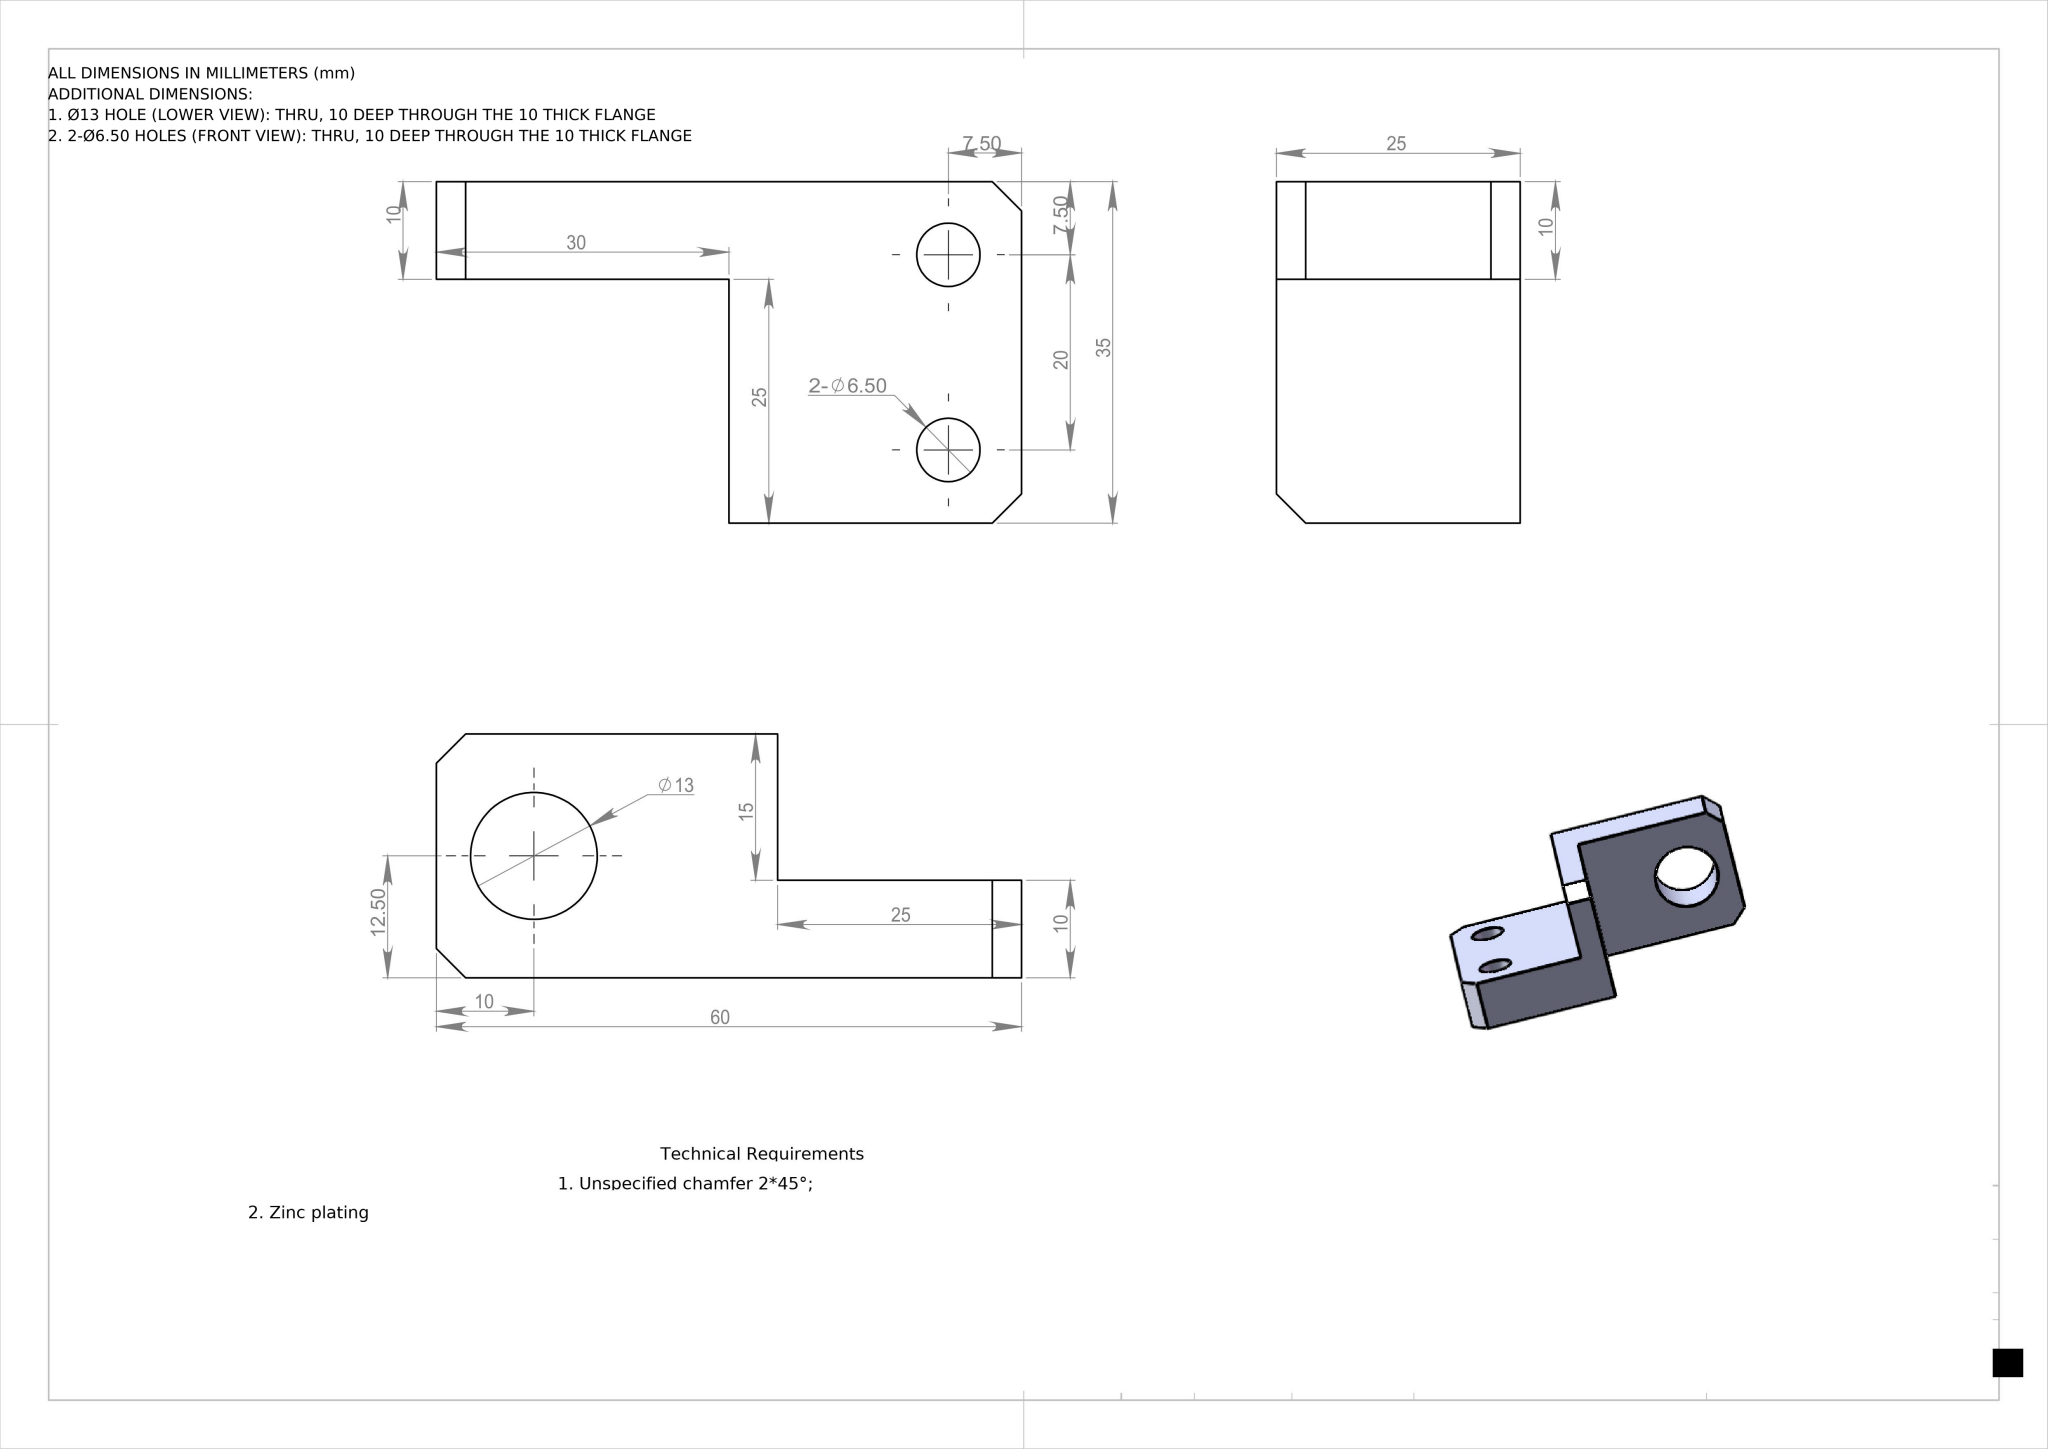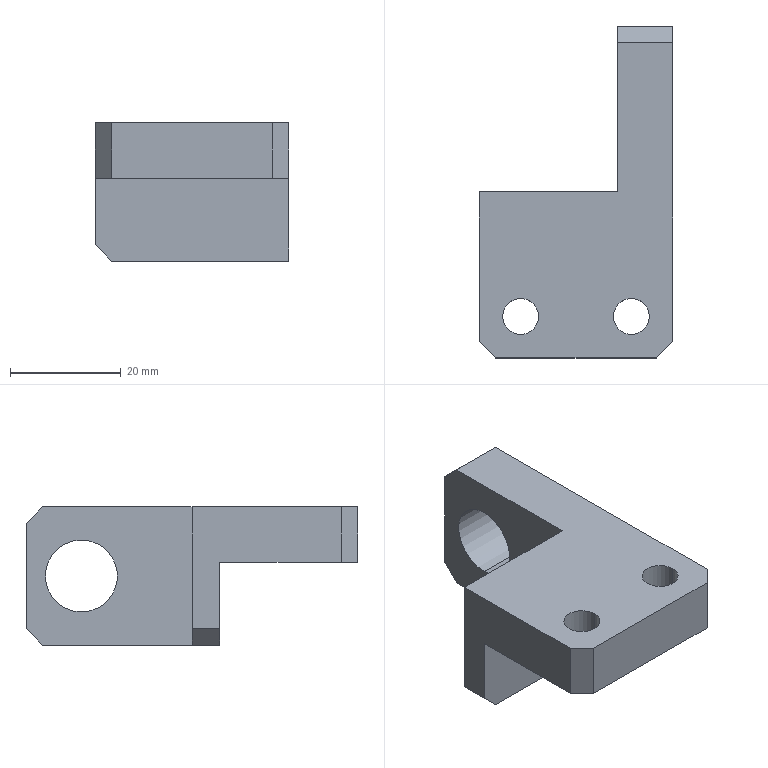Part | NX | mm | 1 solid | 21 faces | box 35 x 60 x 25 mm | volume 18432 mm3 | plane 15 | cylinder 6 | commonest cylinder face diameters 6.5 x4 13 x2
STEP:
#1=COLOUR_RGB('',0.7961,0.8235,0.9373);
#2=FILL_AREA_STYLE_COLOUR('',#1);
#3=FILL_AREA_STYLE('',(#2));
#4=SURFACE_STYLE_FILL_AREA(#3);
#5=SURFACE_SIDE_STYLE('',(#4));
#6=SURFACE_STYLE_USAGE(.BOTH.,#5);
#7=PRESENTATION_STYLE_ASSIGNMENT((#6));
#8=CARTESIAN_POINT('',(-13.25,-22.5,15.));
#9=VERTEX_POINT('',#8);
#10=CARTESIAN_POINT('',(-6.75,-22.5,15.));
#11=VERTEX_POINT('',#10);
#12=CARTESIAN_POINT('',(-10.,-22.5,15.));
#13=DIRECTION('',(0.,0.,1.));
#14=DIRECTION('',(1.,0.,0.));
#15=AXIS2_PLACEMENT_3D('',#12,#13,#14);
#16=CIRCLE('',#15,3.25);
#17=EDGE_CURVE('',#9,#11,#16,.T.);
#18=ORIENTED_EDGE('',*,*,#17,.F.);
#19=CARTESIAN_POINT('',(-13.25,-22.5,25.));
#20=VERTEX_POINT('',#19);
#21=CARTESIAN_POINT('',(-13.25,-22.5,0.));
#22=DIRECTION('',(0.,0.,1.));
#23=VECTOR('',#22,1000.);
#24=LINE('',#21,#23);
#25=EDGE_CURVE('',#9,#20,#24,.T.);
#26=ORIENTED_EDGE('',*,*,#25,.T.);
#27=CARTESIAN_POINT('',(-6.75,-22.5,25.));
#28=VERTEX_POINT('',#27);
#29=CARTESIAN_POINT('',(-10.,-22.5,25.));
#30=DIRECTION('',(0.,0.,1.));
#31=DIRECTION('',(1.,0.,0.));
#32=AXIS2_PLACEMENT_3D('',#29,#30,#31);
#33=CIRCLE('',#32,3.25);
#34=EDGE_CURVE('',#20,#28,#33,.T.);
#35=ORIENTED_EDGE('',*,*,#34,.T.);
#36=CARTESIAN_POINT('',(-6.75,-22.5,0.));
#37=DIRECTION('',(0.,0.,1.));
#38=VECTOR('',#37,1000.);
#39=LINE('',#36,#38);
#40=EDGE_CURVE('',#11,#28,#39,.T.);
#41=ORIENTED_EDGE('',*,*,#40,.F.);
#42=EDGE_LOOP('',(#18,#26,#35,#41));
#43=FACE_OUTER_BOUND('',#42,.T.);
#44=CARTESIAN_POINT('',(-10.,-22.5,0.));
#45=DIRECTION('',(0.,0.,1.));
#46=DIRECTION('',(1.,0.,0.));
#47=AXIS2_PLACEMENT_3D('',#44,#45,#46);
#48=CYLINDRICAL_SURFACE('',#47,3.25);
#49=ADVANCED_FACE('',(#43),#48,.F.);
#50=CARTESIAN_POINT('',(6.75,-22.5,15.));
#51=VERTEX_POINT('',#50);
#52=CARTESIAN_POINT('',(13.25,-22.5,15.));
#53=VERTEX_POINT('',#52);
#54=CARTESIAN_POINT('',(10.,-22.5,15.));
#55=DIRECTION('',(0.,0.,1.));
#56=DIRECTION('',(1.,0.,0.));
#57=AXIS2_PLACEMENT_3D('',#54,#55,#56);
#58=CIRCLE('',#57,3.25);
#59=EDGE_CURVE('',#51,#53,#58,.T.);
#60=ORIENTED_EDGE('',*,*,#59,.F.);
#61=CARTESIAN_POINT('',(6.75,-22.5,25.));
#62=VERTEX_POINT('',#61);
#63=CARTESIAN_POINT('',(6.75,-22.5,0.));
#64=DIRECTION('',(0.,0.,1.));
#65=VECTOR('',#64,1000.);
#66=LINE('',#63,#65);
#67=EDGE_CURVE('',#51,#62,#66,.T.);
#68=ORIENTED_EDGE('',*,*,#67,.T.);
#69=CARTESIAN_POINT('',(13.25,-22.5,25.));
#70=VERTEX_POINT('',#69);
#71=CARTESIAN_POINT('',(10.,-22.5,25.));
#72=DIRECTION('',(0.,0.,1.));
#73=DIRECTION('',(1.,0.,0.));
#74=AXIS2_PLACEMENT_3D('',#71,#72,#73);
#75=CIRCLE('',#74,3.25);
#76=EDGE_CURVE('',#62,#70,#75,.T.);
#77=ORIENTED_EDGE('',*,*,#76,.T.);
#78=CARTESIAN_POINT('',(13.25,-22.5,0.));
#79=DIRECTION('',(0.,0.,1.));
#80=VECTOR('',#79,1000.);
#81=LINE('',#78,#80);
#82=EDGE_CURVE('',#53,#70,#81,.T.);
#83=ORIENTED_EDGE('',*,*,#82,.F.);
#84=EDGE_LOOP('',(#60,#68,#77,#83));
#85=FACE_OUTER_BOUND('',#84,.T.);
#86=CARTESIAN_POINT('',(10.,-22.5,0.));
#87=DIRECTION('',(0.,0.,1.));
#88=DIRECTION('',(1.,0.,0.));
#89=AXIS2_PLACEMENT_3D('',#86,#87,#88);
#90=CYLINDRICAL_SURFACE('',#89,3.25);
#91=ADVANCED_FACE('',(#85),#90,.F.);
#92=CARTESIAN_POINT('',(17.5,20.,6.));
#93=VERTEX_POINT('',#92);
#94=CARTESIAN_POINT('',(17.5,20.,19.));
#95=VERTEX_POINT('',#94);
#96=CARTESIAN_POINT('',(17.5,20.,12.5));
#97=DIRECTION('',(-1.,0.,0.));
#98=DIRECTION('',(0.,0.,1.));
#99=AXIS2_PLACEMENT_3D('',#96,#97,#98);
#100=CIRCLE('',#99,6.5);
#101=EDGE_CURVE('',#93,#95,#100,.T.);
#102=ORIENTED_EDGE('',*,*,#101,.F.);
#103=CARTESIAN_POINT('',(7.5,20.,6.));
#104=VERTEX_POINT('',#103);
#105=CARTESIAN_POINT('',(17.5,20.,6.));
#106=DIRECTION('',(-1.,0.,0.));
#107=VECTOR('',#106,1000.);
#108=LINE('',#105,#107);
#109=EDGE_CURVE('',#93,#104,#108,.T.);
#110=ORIENTED_EDGE('',*,*,#109,.T.);
#111=CARTESIAN_POINT('',(7.5,20.,19.));
#112=VERTEX_POINT('',#111);
#113=CARTESIAN_POINT('',(7.5,20.,12.5));
#114=DIRECTION('',(-1.,-0.,0.));
#115=DIRECTION('',(-0.,1.,0.));
#116=AXIS2_PLACEMENT_3D('',#113,#114,#115);
#117=CIRCLE('',#116,6.5);
#118=EDGE_CURVE('',#104,#112,#117,.T.);
#119=ORIENTED_EDGE('',*,*,#118,.T.);
#120=CARTESIAN_POINT('',(17.5,20.,19.));
#121=DIRECTION('',(-1.,0.,0.));
#122=VECTOR('',#121,1000.);
#123=LINE('',#120,#122);
#124=EDGE_CURVE('',#95,#112,#123,.T.);
#125=ORIENTED_EDGE('',*,*,#124,.F.);
#126=EDGE_LOOP('',(#102,#110,#119,#125));
#127=FACE_OUTER_BOUND('',#126,.T.);
#128=CARTESIAN_POINT('',(17.5,20.,12.5));
#129=DIRECTION('',(-1.,0.,0.));
#130=DIRECTION('',(0.,0.,1.));
#131=AXIS2_PLACEMENT_3D('',#128,#129,#130);
#132=CYLINDRICAL_SURFACE('',#131,6.5);
#133=ADVANCED_FACE('',(#127),#132,.F.);
#134=CARTESIAN_POINT('',(17.5,20.,12.5));
#135=DIRECTION('',(-1.,0.,0.));
#136=DIRECTION('',(0.,0.,1.));
#137=AXIS2_PLACEMENT_3D('',#134,#135,#136);
#138=CIRCLE('',#137,6.5);
#139=EDGE_CURVE('',#95,#93,#138,.T.);
#140=ORIENTED_EDGE('',*,*,#139,.T.);
#141=ORIENTED_EDGE('',*,*,#101,.T.);
#142=EDGE_LOOP('',(#140,#141));
#143=FACE_BOUND('',#142,.T.);
#144=CARTESIAN_POINT('',(17.5,-5.,0.));
#145=VERTEX_POINT('',#144);
#146=CARTESIAN_POINT('',(17.5,27.,0.));
#147=VERTEX_POINT('',#146);
#148=CARTESIAN_POINT('',(17.5,-30.,0.));
#149=DIRECTION('',(0.,1.,0.));
#150=VECTOR('',#149,1000.);
#151=LINE('',#148,#150);
#152=EDGE_CURVE('',#145,#147,#151,.T.);
#153=ORIENTED_EDGE('',*,*,#152,.T.);
#154=CARTESIAN_POINT('',(17.5,30.,3.));
#155=VERTEX_POINT('',#154);
#156=CARTESIAN_POINT('',(17.5,30.,3.));
#157=DIRECTION('',(0.,0.7071,0.7071));
#158=VECTOR('',#157,1000.);
#159=LINE('',#156,#158);
#160=EDGE_CURVE('',#147,#155,#159,.T.);
#161=ORIENTED_EDGE('',*,*,#160,.T.);
#162=CARTESIAN_POINT('',(17.5,30.,22.));
#163=VERTEX_POINT('',#162);
#164=CARTESIAN_POINT('',(17.5,30.,25.));
#165=DIRECTION('',(0.,0.,-1.));
#166=VECTOR('',#165,1000.);
#167=LINE('',#164,#166);
#168=EDGE_CURVE('',#163,#155,#167,.T.);
#169=ORIENTED_EDGE('',*,*,#168,.F.);
#170=CARTESIAN_POINT('',(17.5,27.,25.));
#171=VERTEX_POINT('',#170);
#172=CARTESIAN_POINT('',(17.5,27.,25.));
#173=DIRECTION('',(0.,-0.7071,0.7071));
#174=VECTOR('',#173,1000.);
#175=LINE('',#172,#174);
#176=EDGE_CURVE('',#163,#171,#175,.T.);
#177=ORIENTED_EDGE('',*,*,#176,.T.);
#178=CARTESIAN_POINT('',(17.5,-27.,25.));
#179=VERTEX_POINT('',#178);
#180=CARTESIAN_POINT('',(17.5,-30.,25.));
#181=DIRECTION('',(0.,1.,0.));
#182=VECTOR('',#181,1000.);
#183=LINE('',#180,#182);
#184=EDGE_CURVE('',#179,#171,#183,.T.);
#185=ORIENTED_EDGE('',*,*,#184,.F.);
#186=CARTESIAN_POINT('',(17.5,-27.,15.));
#187=VERTEX_POINT('',#186);
#188=CARTESIAN_POINT('',(17.5,-27.,25.));
#189=DIRECTION('',(0.,0.,-1.));
#190=VECTOR('',#189,1000.);
#191=LINE('',#188,#190);
#192=EDGE_CURVE('',#179,#187,#191,.T.);
#193=ORIENTED_EDGE('',*,*,#192,.T.);
#194=CARTESIAN_POINT('',(17.5,-5.,15.));
#195=VERTEX_POINT('',#194);
#196=CARTESIAN_POINT('',(17.5,-30.,15.));
#197=DIRECTION('',(0.,1.,0.));
#198=VECTOR('',#197,1000.);
#199=LINE('',#196,#198);
#200=EDGE_CURVE('',#187,#195,#199,.T.);
#201=ORIENTED_EDGE('',*,*,#200,.T.);
#202=CARTESIAN_POINT('',(17.5,-5.,0.));
#203=DIRECTION('',(0.,0.,-1.));
#204=VECTOR('',#203,1000.);
#205=LINE('',#202,#204);
#206=EDGE_CURVE('',#195,#145,#205,.T.);
#207=ORIENTED_EDGE('',*,*,#206,.T.);
#208=EDGE_LOOP('',(#153,#161,#169,#177,#185,#193,#201,#207));
#209=FACE_OUTER_BOUND('',#208,.T.);
#210=CARTESIAN_POINT('',(17.5,-30.,25.));
#211=DIRECTION('',(-1.,0.,0.));
#212=DIRECTION('',(0.,0.,1.));
#213=AXIS2_PLACEMENT_3D('',#210,#211,#212);
#214=PLANE('',#213);
#215=ADVANCED_FACE('',(#143,#209),#214,.F.);
#216=ORIENTED_EDGE('',*,*,#168,.T.);
#217=CARTESIAN_POINT('',(7.5,30.,3.));
#218=VERTEX_POINT('',#217);
#219=CARTESIAN_POINT('',(7.5,30.,3.));
#220=DIRECTION('',(-1.,0.,0.));
#221=VECTOR('',#220,1000.);
#222=LINE('',#219,#221);
#223=EDGE_CURVE('',#155,#218,#222,.T.);
#224=ORIENTED_EDGE('',*,*,#223,.T.);
#225=CARTESIAN_POINT('',(7.5,30.,22.));
#226=VERTEX_POINT('',#225);
#227=CARTESIAN_POINT('',(7.5,30.,0.));
#228=DIRECTION('',(0.,0.,1.));
#229=VECTOR('',#228,1000.);
#230=LINE('',#227,#229);
#231=EDGE_CURVE('',#218,#226,#230,.T.);
#232=ORIENTED_EDGE('',*,*,#231,.T.);
#233=CARTESIAN_POINT('',(-17.5,30.,22.));
#234=DIRECTION('',(1.,0.,0.));
#235=VECTOR('',#234,1000.);
#236=LINE('',#233,#235);
#237=EDGE_CURVE('',#226,#163,#236,.T.);
#238=ORIENTED_EDGE('',*,*,#237,.T.);
#239=EDGE_LOOP('',(#216,#224,#232,#238));
#240=FACE_OUTER_BOUND('',#239,.T.);
#241=CARTESIAN_POINT('',(-17.5,30.,25.));
#242=DIRECTION('',(0.,-1.,0.));
#243=DIRECTION('',(0.,0.,-1.));
#244=AXIS2_PLACEMENT_3D('',#241,#242,#243);
#245=PLANE('',#244);
#246=ADVANCED_FACE('',(#240),#245,.F.);
#247=CARTESIAN_POINT('',(-17.5,-27.,15.));
#248=VERTEX_POINT('',#247);
#249=CARTESIAN_POINT('',(-17.5,-5.,15.));
#250=VERTEX_POINT('',#249);
#251=CARTESIAN_POINT('',(-17.5,-30.,15.));
#252=DIRECTION('',(0.,1.,0.));
#253=VECTOR('',#252,1000.);
#254=LINE('',#251,#253);
#255=EDGE_CURVE('',#248,#250,#254,.T.);
#256=ORIENTED_EDGE('',*,*,#255,.F.);
#257=CARTESIAN_POINT('',(-17.5,-27.,25.));
#258=VERTEX_POINT('',#257);
#259=CARTESIAN_POINT('',(-17.5,-27.,25.));
#260=DIRECTION('',(0.,0.,1.));
#261=VECTOR('',#260,1000.);
#262=LINE('',#259,#261);
#263=EDGE_CURVE('',#248,#258,#262,.T.);
#264=ORIENTED_EDGE('',*,*,#263,.T.);
#265=CARTESIAN_POINT('',(-17.5,0.,25.));
#266=VERTEX_POINT('',#265);
#267=CARTESIAN_POINT('',(-17.5,-30.,25.));
#268=DIRECTION('',(0.,-1.,0.));
#269=VECTOR('',#268,1000.);
#270=LINE('',#267,#269);
#271=EDGE_CURVE('',#266,#258,#270,.T.);
#272=ORIENTED_EDGE('',*,*,#271,.F.);
#273=CARTESIAN_POINT('',(-17.5,0.,3.));
#274=VERTEX_POINT('',#273);
#275=CARTESIAN_POINT('',(-17.5,0.,0.));
#276=DIRECTION('',(0.,0.,1.));
#277=VECTOR('',#276,1000.);
#278=LINE('',#275,#277);
#279=EDGE_CURVE('',#274,#266,#278,.T.);
#280=ORIENTED_EDGE('',*,*,#279,.F.);
#281=CARTESIAN_POINT('',(-17.5,-5.,3.));
#282=VERTEX_POINT('',#281);
#283=CARTESIAN_POINT('',(-17.5,-5.,3.));
#284=DIRECTION('',(0.,-1.,0.));
#285=VECTOR('',#284,1000.);
#286=LINE('',#283,#285);
#287=EDGE_CURVE('',#274,#282,#286,.T.);
#288=ORIENTED_EDGE('',*,*,#287,.T.);
#289=CARTESIAN_POINT('',(-17.5,-5.,0.));
#290=DIRECTION('',(0.,0.,-1.));
#291=VECTOR('',#290,1000.);
#292=LINE('',#289,#291);
#293=EDGE_CURVE('',#250,#282,#292,.T.);
#294=ORIENTED_EDGE('',*,*,#293,.F.);
#295=EDGE_LOOP('',(#256,#264,#272,#280,#288,#294));
#296=FACE_OUTER_BOUND('',#295,.T.);
#297=CARTESIAN_POINT('',(-17.5,-30.,25.));
#298=DIRECTION('',(1.,0.,0.));
#299=DIRECTION('',(0.,0.,-1.));
#300=AXIS2_PLACEMENT_3D('',#297,#298,#299);
#301=PLANE('',#300);
#302=ADVANCED_FACE('',(#296),#301,.F.);
#303=CARTESIAN_POINT('',(14.5,-30.,15.));
#304=VERTEX_POINT('',#303);
#305=CARTESIAN_POINT('',(-14.5,-30.,15.));
#306=VERTEX_POINT('',#305);
#307=CARTESIAN_POINT('',(17.5,-30.,15.));
#308=DIRECTION('',(-1.,0.,0.));
#309=VECTOR('',#308,1000.);
#310=LINE('',#307,#309);
#311=EDGE_CURVE('',#304,#306,#310,.T.);
#312=ORIENTED_EDGE('',*,*,#311,.F.);
#313=CARTESIAN_POINT('',(14.5,-30.,25.));
#314=VERTEX_POINT('',#313);
#315=CARTESIAN_POINT('',(14.5,-30.,25.));
#316=DIRECTION('',(0.,0.,1.));
#317=VECTOR('',#316,1000.);
#318=LINE('',#315,#317);
#319=EDGE_CURVE('',#304,#314,#318,.T.);
#320=ORIENTED_EDGE('',*,*,#319,.T.);
#321=CARTESIAN_POINT('',(-14.5,-30.,25.));
#322=VERTEX_POINT('',#321);
#323=CARTESIAN_POINT('',(-17.5,-30.,25.));
#324=DIRECTION('',(1.,0.,0.));
#325=VECTOR('',#324,1000.);
#326=LINE('',#323,#325);
#327=EDGE_CURVE('',#322,#314,#326,.T.);
#328=ORIENTED_EDGE('',*,*,#327,.F.);
#329=CARTESIAN_POINT('',(-14.5,-30.,25.));
#330=DIRECTION('',(0.,0.,-1.));
#331=VECTOR('',#330,1000.);
#332=LINE('',#329,#331);
#333=EDGE_CURVE('',#322,#306,#332,.T.);
#334=ORIENTED_EDGE('',*,*,#333,.T.);
#335=EDGE_LOOP('',(#312,#320,#328,#334));
#336=FACE_OUTER_BOUND('',#335,.T.);
#337=CARTESIAN_POINT('',(-17.5,-30.,25.));
#338=DIRECTION('',(0.,1.,0.));
#339=DIRECTION('',(0.,0.,1.));
#340=AXIS2_PLACEMENT_3D('',#337,#338,#339);
#341=PLANE('',#340);
#342=ADVANCED_FACE('',(#336),#341,.F.);
#343=CARTESIAN_POINT('',(-10.,-22.5,25.));
#344=DIRECTION('',(0.,0.,1.));
#345=DIRECTION('',(1.,0.,0.));
#346=AXIS2_PLACEMENT_3D('',#343,#344,#345);
#347=CIRCLE('',#346,3.25);
#348=EDGE_CURVE('',#28,#20,#347,.T.);
#349=ORIENTED_EDGE('',*,*,#348,.F.);
#350=ORIENTED_EDGE('',*,*,#34,.F.);
#351=EDGE_LOOP('',(#349,#350));
#352=FACE_BOUND('',#351,.T.);
#353=CARTESIAN_POINT('',(10.,-22.5,25.));
#354=DIRECTION('',(0.,0.,1.));
#355=DIRECTION('',(1.,0.,0.));
#356=AXIS2_PLACEMENT_3D('',#353,#354,#355);
#357=CIRCLE('',#356,3.25);
#358=EDGE_CURVE('',#70,#62,#357,.T.);
#359=ORIENTED_EDGE('',*,*,#358,.F.);
#360=ORIENTED_EDGE('',*,*,#76,.F.);
#361=EDGE_LOOP('',(#359,#360));
#362=FACE_BOUND('',#361,.T.);
#363=ORIENTED_EDGE('',*,*,#184,.T.);
#364=CARTESIAN_POINT('',(7.5,27.,25.));
#365=VERTEX_POINT('',#364);
#366=CARTESIAN_POINT('',(0.,27.,25.));
#367=DIRECTION('',(-1.,0.,0.));
#368=VECTOR('',#367,1000.);
#369=LINE('',#366,#368);
#370=EDGE_CURVE('',#171,#365,#369,.T.);
#371=ORIENTED_EDGE('',*,*,#370,.T.);
#372=CARTESIAN_POINT('',(7.5,0.,25.));
#373=VERTEX_POINT('',#372);
#374=CARTESIAN_POINT('',(7.5,30.,25.));
#375=DIRECTION('',(-0.,1.,0.));
#376=VECTOR('',#375,1000.);
#377=LINE('',#374,#376);
#378=EDGE_CURVE('',#373,#365,#377,.T.);
#379=ORIENTED_EDGE('',*,*,#378,.F.);
#380=CARTESIAN_POINT('',(-17.5,0.,25.));
#381=DIRECTION('',(1.,0.,0.));
#382=VECTOR('',#381,1000.);
#383=LINE('',#380,#382);
#384=EDGE_CURVE('',#266,#373,#383,.T.);
#385=ORIENTED_EDGE('',*,*,#384,.F.);
#386=ORIENTED_EDGE('',*,*,#271,.T.);
#387=CARTESIAN_POINT('',(-14.5,-30.,25.));
#388=DIRECTION('',(0.7071,-0.7071,0.));
#389=VECTOR('',#388,1000.);
#390=LINE('',#387,#389);
#391=EDGE_CURVE('',#258,#322,#390,.T.);
#392=ORIENTED_EDGE('',*,*,#391,.T.);
#393=ORIENTED_EDGE('',*,*,#327,.T.);
#394=CARTESIAN_POINT('',(17.5,-27.,25.));
#395=DIRECTION('',(0.7071,0.7071,0.));
#396=VECTOR('',#395,1000.);
#397=LINE('',#394,#396);
#398=EDGE_CURVE('',#314,#179,#397,.T.);
#399=ORIENTED_EDGE('',*,*,#398,.T.);
#400=EDGE_LOOP('',(#363,#371,#379,#385,#386,#392,#393,#399));
#401=FACE_OUTER_BOUND('',#400,.T.);
#402=CARTESIAN_POINT('',(0.,0.,25.));
#403=DIRECTION('',(0.,0.,-1.));
#404=DIRECTION('',(-1.,0.,0.));
#405=AXIS2_PLACEMENT_3D('',#402,#403,#404);
#406=PLANE('',#405);
#407=ADVANCED_FACE('',(#352,#362,#401),#406,.F.);
#408=CARTESIAN_POINT('',(7.5,0.,0.));
#409=VERTEX_POINT('',#408);
#410=CARTESIAN_POINT('',(7.5,27.,0.));
#411=VERTEX_POINT('',#410);
#412=CARTESIAN_POINT('',(7.5,30.,0.));
#413=DIRECTION('',(-0.,1.,0.));
#414=VECTOR('',#413,1000.);
#415=LINE('',#412,#414);
#416=EDGE_CURVE('',#409,#411,#415,.T.);
#417=ORIENTED_EDGE('',*,*,#416,.T.);
#418=CARTESIAN_POINT('',(17.5,27.,0.));
#419=DIRECTION('',(1.,0.,0.));
#420=VECTOR('',#419,1000.);
#421=LINE('',#418,#420);
#422=EDGE_CURVE('',#411,#147,#421,.T.);
#423=ORIENTED_EDGE('',*,*,#422,.T.);
#424=ORIENTED_EDGE('',*,*,#152,.F.);
#425=CARTESIAN_POINT('',(-14.5,-5.,0.));
#426=VERTEX_POINT('',#425);
#427=CARTESIAN_POINT('',(17.5,-5.,0.));
#428=DIRECTION('',(-1.,0.,0.));
#429=VECTOR('',#428,1000.);
#430=LINE('',#427,#429);
#431=EDGE_CURVE('',#145,#426,#430,.T.);
#432=ORIENTED_EDGE('',*,*,#431,.T.);
#433=CARTESIAN_POINT('',(-14.5,0.,0.));
#434=VERTEX_POINT('',#433);
#435=CARTESIAN_POINT('',(-14.5,0.,0.));
#436=DIRECTION('',(0.,1.,0.));
#437=VECTOR('',#436,1000.);
#438=LINE('',#435,#437);
#439=EDGE_CURVE('',#426,#434,#438,.T.);
#440=ORIENTED_EDGE('',*,*,#439,.T.);
#441=CARTESIAN_POINT('',(-17.5,0.,0.));
#442=DIRECTION('',(1.,0.,0.));
#443=VECTOR('',#442,1000.);
#444=LINE('',#441,#443);
#445=EDGE_CURVE('',#434,#409,#444,.T.);
#446=ORIENTED_EDGE('',*,*,#445,.T.);
#447=EDGE_LOOP('',(#417,#423,#424,#432,#440,#446));
#448=FACE_OUTER_BOUND('',#447,.T.);
#449=CARTESIAN_POINT('',(0.,0.,0.));
#450=DIRECTION('',(0.,0.,-1.));
#451=DIRECTION('',(-1.,0.,0.));
#452=AXIS2_PLACEMENT_3D('',#449,#450,#451);
#453=PLANE('',#452);
#454=ADVANCED_FACE('',(#448),#453,.T.);
#455=ORIENTED_EDGE('',*,*,#109,.F.);
#456=ORIENTED_EDGE('',*,*,#139,.F.);
#457=ORIENTED_EDGE('',*,*,#124,.T.);
#458=CARTESIAN_POINT('',(7.5,20.,12.5));
#459=DIRECTION('',(-1.,-0.,0.));
#460=DIRECTION('',(-0.,1.,0.));
#461=AXIS2_PLACEMENT_3D('',#458,#459,#460);
#462=CIRCLE('',#461,6.5);
#463=EDGE_CURVE('',#112,#104,#462,.T.);
#464=ORIENTED_EDGE('',*,*,#463,.T.);
#465=EDGE_LOOP('',(#455,#456,#457,#464));
#466=FACE_OUTER_BOUND('',#465,.T.);
#467=CARTESIAN_POINT('',(17.5,20.,12.5));
#468=DIRECTION('',(-1.,0.,0.));
#469=DIRECTION('',(0.,0.,1.));
#470=AXIS2_PLACEMENT_3D('',#467,#468,#469);
#471=CYLINDRICAL_SURFACE('',#470,6.5);
#472=ADVANCED_FACE('',(#466),#471,.F.);
#473=ORIENTED_EDGE('',*,*,#293,.T.);
#474=CARTESIAN_POINT('',(-17.5,-5.,3.));
#475=DIRECTION('',(0.7071,0.,-0.7071));
#476=VECTOR('',#475,1000.);
#477=LINE('',#474,#476);
#478=EDGE_CURVE('',#282,#426,#477,.T.);
#479=ORIENTED_EDGE('',*,*,#478,.T.);
#480=ORIENTED_EDGE('',*,*,#431,.F.);
#481=ORIENTED_EDGE('',*,*,#206,.F.);
#482=CARTESIAN_POINT('',(17.5,-5.,15.));
#483=DIRECTION('',(-1.,0.,0.));
#484=VECTOR('',#483,1000.);
#485=LINE('',#482,#484);
#486=EDGE_CURVE('',#195,#250,#485,.T.);
#487=ORIENTED_EDGE('',*,*,#486,.T.);
#488=EDGE_LOOP('',(#473,#479,#480,#481,#487));
#489=FACE_OUTER_BOUND('',#488,.T.);
#490=CARTESIAN_POINT('',(17.5,-5.,0.));
#491=DIRECTION('',(0.,1.,0.));
#492=DIRECTION('',(0.,0.,1.));
#493=AXIS2_PLACEMENT_3D('',#490,#491,#492);
#494=PLANE('',#493);
#495=ADVANCED_FACE('',(#489),#494,.F.);
#496=CARTESIAN_POINT('',(-10.,-22.5,15.));
#497=DIRECTION('',(0.,0.,1.));
#498=DIRECTION('',(1.,0.,0.));
#499=AXIS2_PLACEMENT_3D('',#496,#497,#498);
#500=CIRCLE('',#499,3.25);
#501=EDGE_CURVE('',#11,#9,#500,.T.);
#502=ORIENTED_EDGE('',*,*,#501,.T.);
#503=ORIENTED_EDGE('',*,*,#17,.T.);
#504=EDGE_LOOP('',(#502,#503));
#505=FACE_BOUND('',#504,.T.);
#506=CARTESIAN_POINT('',(10.,-22.5,15.));
#507=DIRECTION('',(0.,0.,1.));
#508=DIRECTION('',(1.,0.,0.));
#509=AXIS2_PLACEMENT_3D('',#506,#507,#508);
#510=CIRCLE('',#509,3.25);
#511=EDGE_CURVE('',#53,#51,#510,.T.);
#512=ORIENTED_EDGE('',*,*,#511,.T.);
#513=ORIENTED_EDGE('',*,*,#59,.T.);
#514=EDGE_LOOP('',(#512,#513));
#515=FACE_BOUND('',#514,.T.);
#516=ORIENTED_EDGE('',*,*,#200,.F.);
#517=CARTESIAN_POINT('',(17.5,-27.,15.));
#518=DIRECTION('',(-0.7071,-0.7071,0.));
#519=VECTOR('',#518,1000.);
#520=LINE('',#517,#519);
#521=EDGE_CURVE('',#187,#304,#520,.T.);
#522=ORIENTED_EDGE('',*,*,#521,.T.);
#523=ORIENTED_EDGE('',*,*,#311,.T.);
#524=CARTESIAN_POINT('',(-14.5,-30.,15.));
#525=DIRECTION('',(-0.7071,0.7071,0.));
#526=VECTOR('',#525,1000.);
#527=LINE('',#524,#526);
#528=EDGE_CURVE('',#306,#248,#527,.T.);
#529=ORIENTED_EDGE('',*,*,#528,.T.);
#530=ORIENTED_EDGE('',*,*,#255,.T.);
#531=ORIENTED_EDGE('',*,*,#486,.F.);
#532=EDGE_LOOP('',(#516,#522,#523,#529,#530,#531));
#533=FACE_OUTER_BOUND('',#532,.T.);
#534=CARTESIAN_POINT('',(17.5,-30.,15.));
#535=DIRECTION('',(0.,0.,1.));
#536=DIRECTION('',(1.,0.,0.));
#537=AXIS2_PLACEMENT_3D('',#534,#535,#536);
#538=PLANE('',#537);
#539=ADVANCED_FACE('',(#505,#515,#533),#538,.F.);
#540=ORIENTED_EDGE('',*,*,#231,.F.);
#541=CARTESIAN_POINT('',(7.5,30.,3.));
#542=DIRECTION('',(0.,-0.7071,-0.7071));
#543=VECTOR('',#542,1000.);
#544=LINE('',#541,#543);
#545=EDGE_CURVE('',#218,#411,#544,.T.);
#546=ORIENTED_EDGE('',*,*,#545,.T.);
#547=ORIENTED_EDGE('',*,*,#416,.F.);
#548=CARTESIAN_POINT('',(7.5,0.,0.));
#549=DIRECTION('',(0.,0.,1.));
#550=VECTOR('',#549,1000.);
#551=LINE('',#548,#550);
#552=EDGE_CURVE('',#409,#373,#551,.T.);
#553=ORIENTED_EDGE('',*,*,#552,.T.);
#554=ORIENTED_EDGE('',*,*,#378,.T.);
#555=CARTESIAN_POINT('',(7.5,27.,25.));
#556=DIRECTION('',(-0.,0.7071,-0.7071));
#557=VECTOR('',#556,1000.);
#558=LINE('',#555,#557);
#559=EDGE_CURVE('',#365,#226,#558,.T.);
#560=ORIENTED_EDGE('',*,*,#559,.T.);
#561=EDGE_LOOP('',(#540,#546,#547,#553,#554,#560));
#562=FACE_OUTER_BOUND('',#561,.T.);
#563=ORIENTED_EDGE('',*,*,#463,.F.);
#564=ORIENTED_EDGE('',*,*,#118,.F.);
#565=EDGE_LOOP('',(#563,#564));
#566=FACE_BOUND('',#565,.T.);
#567=CARTESIAN_POINT('',(7.5,30.,0.));
#568=DIRECTION('',(1.,0.,0.));
#569=DIRECTION('',(-0.,1.,0.));
#570=AXIS2_PLACEMENT_3D('',#567,#568,#569);
#571=PLANE('',#570);
#572=ADVANCED_FACE('',(#562,#566),#571,.F.);
#573=ORIENTED_EDGE('',*,*,#445,.F.);
#574=CARTESIAN_POINT('',(-17.5,0.,3.));
#575=DIRECTION('',(-0.7071,0.,0.7071));
#576=VECTOR('',#575,1000.);
#577=LINE('',#574,#576);
#578=EDGE_CURVE('',#434,#274,#577,.T.);
#579=ORIENTED_EDGE('',*,*,#578,.T.);
#580=ORIENTED_EDGE('',*,*,#279,.T.);
#581=ORIENTED_EDGE('',*,*,#384,.T.);
#582=ORIENTED_EDGE('',*,*,#552,.F.);
#583=EDGE_LOOP('',(#573,#579,#580,#581,#582));
#584=FACE_OUTER_BOUND('',#583,.T.);
#585=CARTESIAN_POINT('',(-17.5,0.,0.));
#586=DIRECTION('',(0.,-1.,0.));
#587=DIRECTION('',(0.,0.,-1.));
#588=AXIS2_PLACEMENT_3D('',#585,#586,#587);
#589=PLANE('',#588);
#590=ADVANCED_FACE('',(#584),#589,.F.);
#591=ORIENTED_EDGE('',*,*,#160,.F.);
#592=ORIENTED_EDGE('',*,*,#422,.F.);
#593=ORIENTED_EDGE('',*,*,#545,.F.);
#594=ORIENTED_EDGE('',*,*,#223,.F.);
#595=EDGE_LOOP('',(#591,#592,#593,#594));
#596=FACE_OUTER_BOUND('',#595,.T.);
#597=CARTESIAN_POINT('',(-17.5,30.,3.));
#598=DIRECTION('',(0.,0.7071,-0.7071));
#599=DIRECTION('',(1.,0.,0.));
#600=AXIS2_PLACEMENT_3D('',#597,#598,#599);
#601=PLANE('',#600);
#602=ADVANCED_FACE('',(#596),#601,.T.);
#603=ORIENTED_EDGE('',*,*,#176,.F.);
#604=ORIENTED_EDGE('',*,*,#237,.F.);
#605=ORIENTED_EDGE('',*,*,#559,.F.);
#606=ORIENTED_EDGE('',*,*,#370,.F.);
#607=EDGE_LOOP('',(#603,#604,#605,#606));
#608=FACE_OUTER_BOUND('',#607,.T.);
#609=CARTESIAN_POINT('',(0.,27.,25.));
#610=DIRECTION('',(0.,-0.7071,-0.7071));
#611=DIRECTION('',(-1.,0.,0.));
#612=AXIS2_PLACEMENT_3D('',#609,#610,#611);
#613=PLANE('',#612);
#614=ADVANCED_FACE('',(#608),#613,.F.);
#615=ORIENTED_EDGE('',*,*,#398,.F.);
#616=ORIENTED_EDGE('',*,*,#319,.F.);
#617=ORIENTED_EDGE('',*,*,#521,.F.);
#618=ORIENTED_EDGE('',*,*,#192,.F.);
#619=EDGE_LOOP('',(#615,#616,#617,#618));
#620=FACE_OUTER_BOUND('',#619,.T.);
#621=CARTESIAN_POINT('',(17.5,-27.,25.));
#622=DIRECTION('',(-0.7071,0.7071,0.));
#623=DIRECTION('',(0.,0.,-1.));
#624=AXIS2_PLACEMENT_3D('',#621,#622,#623);
#625=PLANE('',#624);
#626=ADVANCED_FACE('',(#620),#625,.F.);
#627=ORIENTED_EDGE('',*,*,#391,.F.);
#628=ORIENTED_EDGE('',*,*,#263,.F.);
#629=ORIENTED_EDGE('',*,*,#528,.F.);
#630=ORIENTED_EDGE('',*,*,#333,.F.);
#631=EDGE_LOOP('',(#627,#628,#629,#630));
#632=FACE_OUTER_BOUND('',#631,.T.);
#633=CARTESIAN_POINT('',(-14.5,-30.,25.));
#634=DIRECTION('',(0.7071,0.7071,0.));
#635=DIRECTION('',(0.,0.,-1.));
#636=AXIS2_PLACEMENT_3D('',#633,#634,#635);
#637=PLANE('',#636);
#638=ADVANCED_FACE('',(#632),#637,.F.);
#639=ORIENTED_EDGE('',*,*,#578,.F.);
#640=ORIENTED_EDGE('',*,*,#439,.F.);
#641=ORIENTED_EDGE('',*,*,#478,.F.);
#642=ORIENTED_EDGE('',*,*,#287,.F.);
#643=EDGE_LOOP('',(#639,#640,#641,#642));
#644=FACE_OUTER_BOUND('',#643,.T.);
#645=CARTESIAN_POINT('',(-17.5,-30.,3.));
#646=DIRECTION('',(-0.7071,0.,-0.7071));
#647=DIRECTION('',(0.,1.,0.));
#648=AXIS2_PLACEMENT_3D('',#645,#646,#647);
#649=PLANE('',#648);
#650=ADVANCED_FACE('',(#644),#649,.T.);
#651=ORIENTED_EDGE('',*,*,#67,.F.);
#652=ORIENTED_EDGE('',*,*,#511,.F.);
#653=ORIENTED_EDGE('',*,*,#82,.T.);
#654=ORIENTED_EDGE('',*,*,#358,.T.);
#655=EDGE_LOOP('',(#651,#652,#653,#654));
#656=FACE_OUTER_BOUND('',#655,.T.);
#657=CARTESIAN_POINT('',(10.,-22.5,0.));
#658=DIRECTION('',(0.,0.,1.));
#659=DIRECTION('',(1.,0.,0.));
#660=AXIS2_PLACEMENT_3D('',#657,#658,#659);
#661=CYLINDRICAL_SURFACE('',#660,3.25);
#662=ADVANCED_FACE('',(#656),#661,.F.);
#663=ORIENTED_EDGE('',*,*,#25,.F.);
#664=ORIENTED_EDGE('',*,*,#501,.F.);
#665=ORIENTED_EDGE('',*,*,#40,.T.);
#666=ORIENTED_EDGE('',*,*,#348,.T.);
#667=EDGE_LOOP('',(#663,#664,#665,#666));
#668=FACE_OUTER_BOUND('',#667,.T.);
#669=CARTESIAN_POINT('',(-10.,-22.5,0.));
#670=DIRECTION('',(0.,0.,1.));
#671=DIRECTION('',(1.,0.,0.));
#672=AXIS2_PLACEMENT_3D('',#669,#670,#671);
#673=CYLINDRICAL_SURFACE('',#672,3.25);
#674=ADVANCED_FACE('',(#668),#673,.F.);
#675=CLOSED_SHELL('',(#49,#91,#133,#215,#246,#302,#342,#407,#454,#472,#495,#539,#572,#590,#602,#614,#626,#638,#650,#662,#674));
#676=MANIFOLD_SOLID_BREP('',#675);
#677=CARTESIAN_POINT('',(0.,0.,0.));
#678=DIRECTION('',(0.,0.,1.));
#679=DIRECTION('',(1.,0.,0.));
#680=AXIS2_PLACEMENT_3D('',#677,#678,#679);
#681=(LENGTH_UNIT()NAMED_UNIT(*)SI_UNIT(.MILLI.,.METRE.));
#682=UNCERTAINTY_MEASURE_WITH_UNIT(LENGTH_MEASURE(0.00001),#681,'','');
#683=(NAMED_UNIT(*)PLANE_ANGLE_UNIT()SI_UNIT($,.RADIAN.));
#684=(NAMED_UNIT(*)SI_UNIT($,.STERADIAN.)SOLID_ANGLE_UNIT());
#685=(GEOMETRIC_REPRESENTATION_CONTEXT(3)GLOBAL_UNCERTAINTY_ASSIGNED_CONTEXT((#682))GLOBAL_UNIT_ASSIGNED_CONTEXT((#681,#683,#684))REPRESENTATION_CONTEXT('',''));
#686=ADVANCED_BREP_SHAPE_REPRESENTATION('',(#676,#680),#685);
#687=STYLED_ITEM('',(#7),#686);
#688=PRESENTATION_LAYER_ASSIGNMENT('','',(#687));
#689=COLOUR_RGB('',0.7961,0.8235,0.9373);
#690=FILL_AREA_STYLE_COLOUR('',#689);
#691=FILL_AREA_STYLE('',(#690));
#692=SURFACE_STYLE_FILL_AREA(#691);
#693=SURFACE_SIDE_STYLE('',(#692));
#694=SURFACE_STYLE_USAGE(.BOTH.,#693);
#695=PRESENTATION_STYLE_ASSIGNMENT((#694));
#696=STYLED_ITEM('',(#695),#676);
#697=(LENGTH_UNIT()NAMED_UNIT(*)SI_UNIT(.MILLI.,.METRE.));
#698=UNCERTAINTY_MEASURE_WITH_UNIT(LENGTH_MEASURE(0.00001),#697,'','');
#699=(NAMED_UNIT(*)PLANE_ANGLE_UNIT()SI_UNIT($,.RADIAN.));
#700=(NAMED_UNIT(*)SI_UNIT($,.STERADIAN.)SOLID_ANGLE_UNIT());
#701=(GEOMETRIC_REPRESENTATION_CONTEXT(3)GLOBAL_UNCERTAINTY_ASSIGNED_CONTEXT((#698))GLOBAL_UNIT_ASSIGNED_CONTEXT((#697,#699,#700))REPRESENTATION_CONTEXT('',''));
#702=MECHANICAL_DESIGN_GEOMETRIC_PRESENTATION_REPRESENTATION('',(#696),#701);
#703=PRESENTATION_LAYER_ASSIGNMENT('','',(#696));
#704=(LENGTH_UNIT()NAMED_UNIT(*)SI_UNIT(.MILLI.,.METRE.));
#705=UNCERTAINTY_MEASURE_WITH_UNIT(LENGTH_MEASURE(0.00001),#704,'','');
#706=(NAMED_UNIT(*)PLANE_ANGLE_UNIT()SI_UNIT($,.RADIAN.));
#707=(NAMED_UNIT(*)SI_UNIT($,.STERADIAN.)SOLID_ANGLE_UNIT());
#708=(GEOMETRIC_REPRESENTATION_CONTEXT(3)GLOBAL_UNCERTAINTY_ASSIGNED_CONTEXT((#705))GLOBAL_UNIT_ASSIGNED_CONTEXT((#704,#706,#707))REPRESENTATION_CONTEXT('',''));
#709=MECHANICAL_DESIGN_GEOMETRIC_PRESENTATION_REPRESENTATION('',(#687),#708);